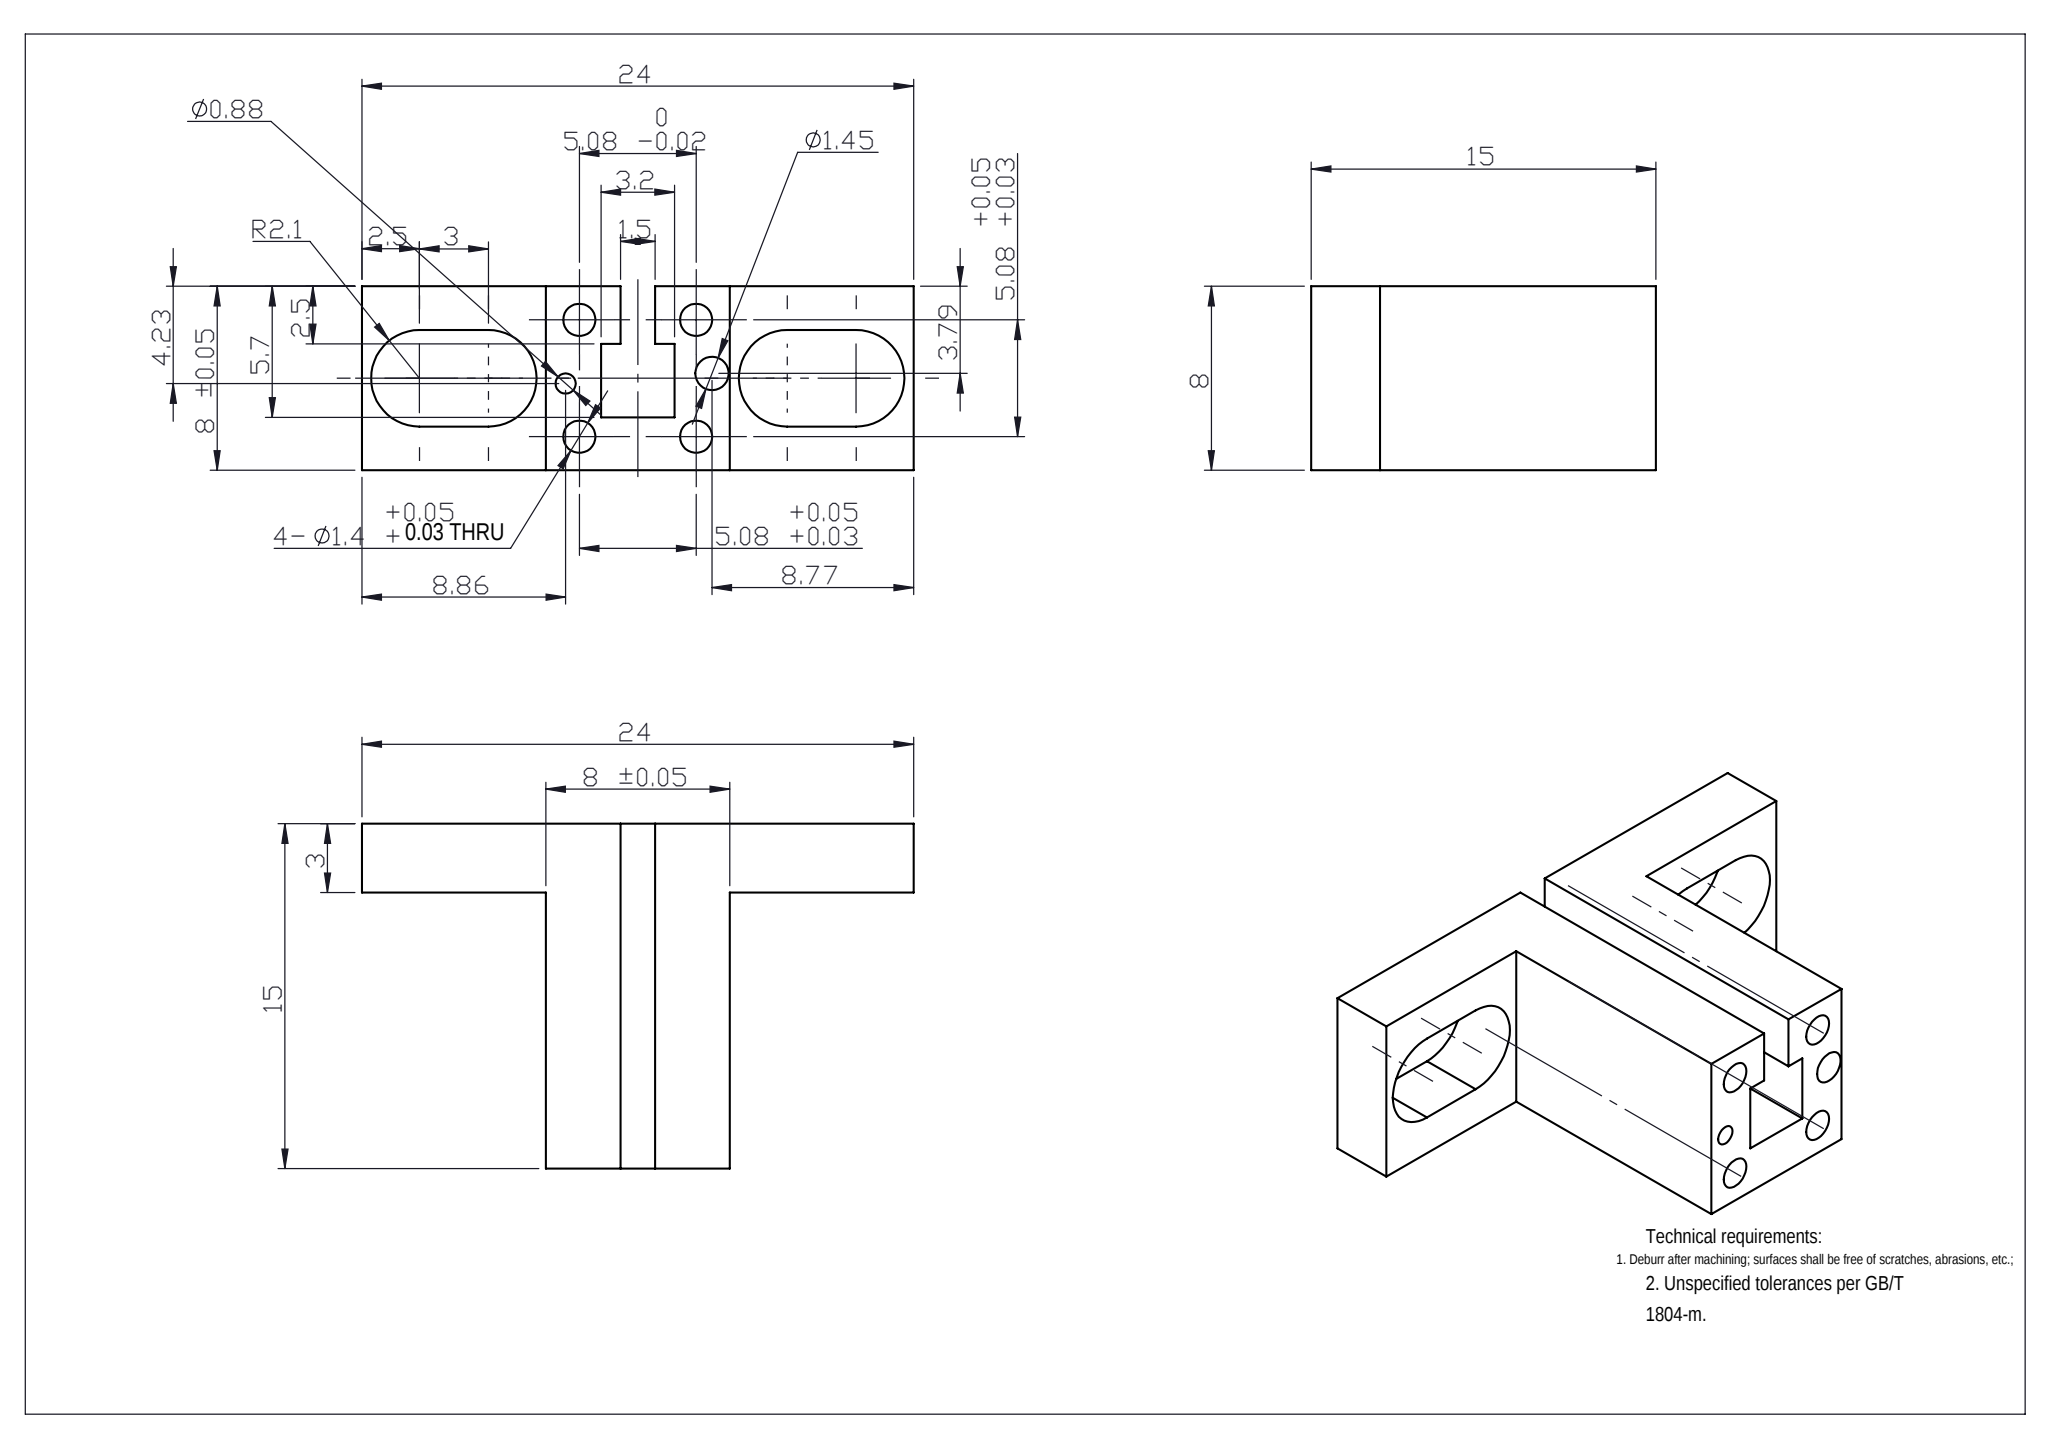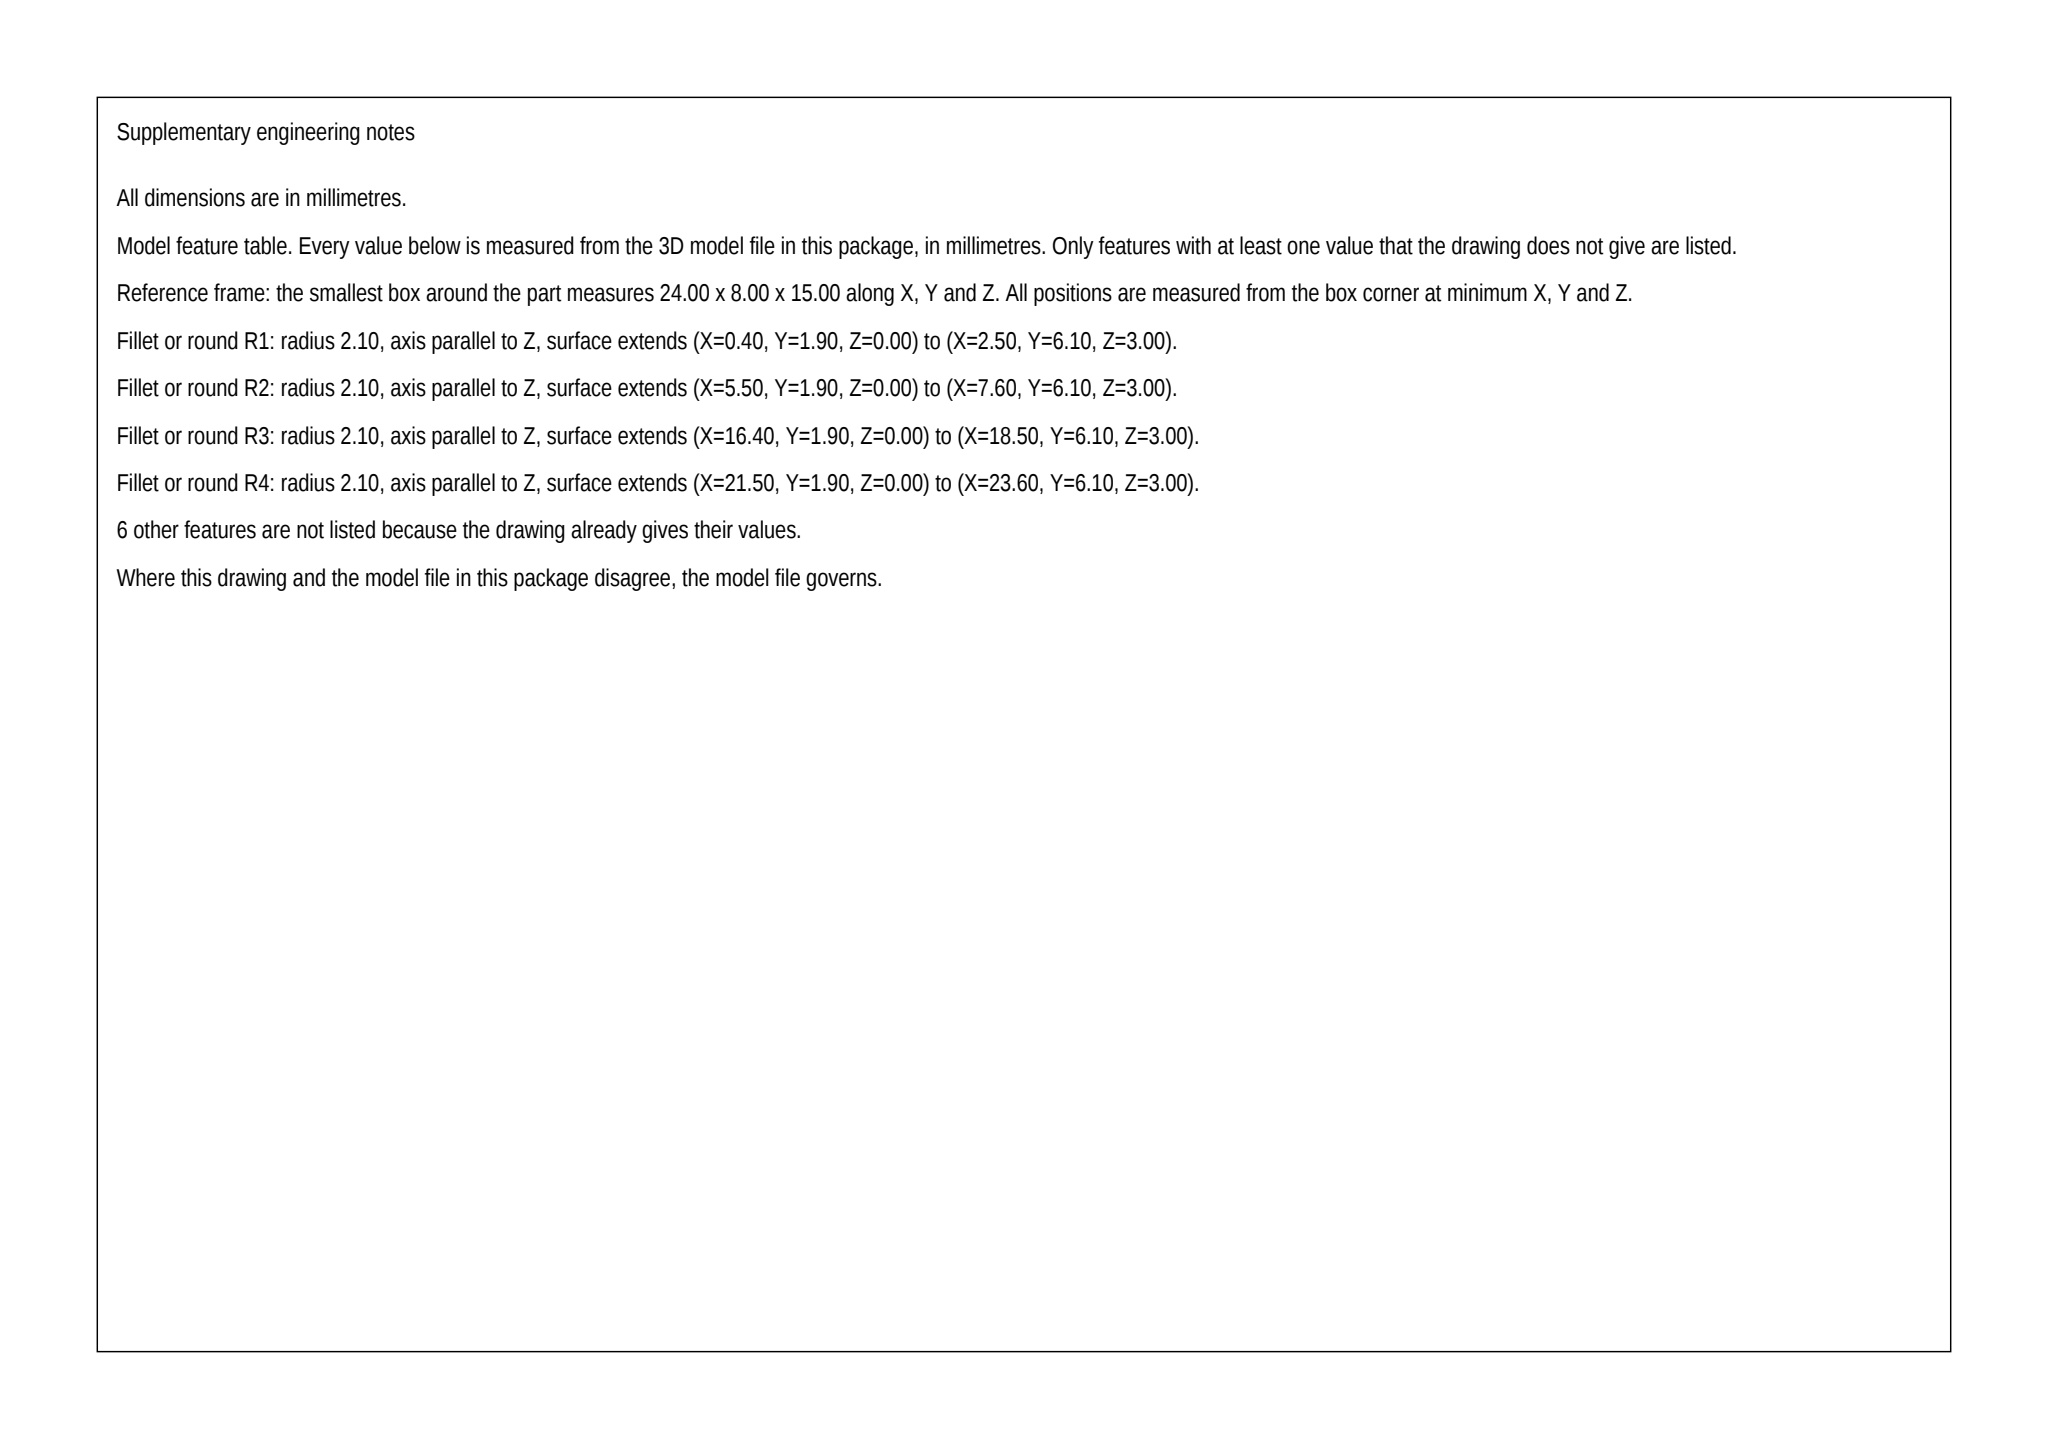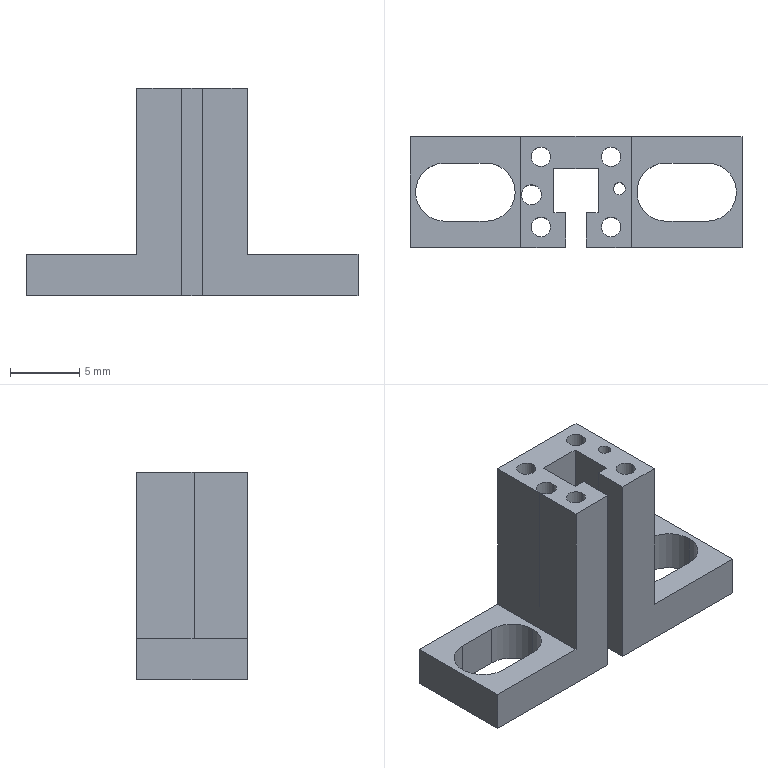Part | SolidWorks | mm | 1 solid | 40 faces | box 24 x 8 x 15 mm | volume 849 mm3 | plane 22 | cylinder 18 | commonest cylinder face diameters 1.4 x8 4.2 x6 0.879 x2 1.45 x2
build123d program:
from build123d import *

# Parameters (mm, degrees)
SKETCH1_W           = 8
SKETCH1_H           = 8
BOSS_EXTRUDE1_DEPTH = 15
SKETCH2_W           = 3
SKETCH2_H           = 8
BOSS_EXTRUDE2_DEPTH = 8
SKETCH3_W           = 3
SKETCH3_H           = 8
BOSS_EXTRUDE3_DEPTH = 8
CUT_EXTRUDE1_DEPTH  = 22.541
SKETCH7_R           = 0.7
CUT_EXTRUDE4_DEPTH  = 24.345
CUT_EXTRUDE5_DEPTH  = 24.345
SKETCH9_R           = 0.4393
SKETCH9_R_2         = 0.7249
CUT_EXTRUDE6_DEPTH  = 17


with BuildPart() as part:
    # Sketch1 → Boss-Extrude1 (new body)
    with BuildSketch(Plane.XY):
        with Locations((4, -4)):
            Rectangle(SKETCH1_W, SKETCH1_H)
    extrude(amount=BOSS_EXTRUDE1_DEPTH)

    # Sketch2 → Boss-Extrude2 (add)
    with BuildSketch(Plane(origin=(8, 0, 0), x_dir=(0, 0, -1), z_dir=(1, 0, 0))):
        with Locations((-1.5, -4)):
            Rectangle(SKETCH2_W, SKETCH2_H)
    extrude(amount=BOSS_EXTRUDE2_DEPTH)

    # Sketch3 → Boss-Extrude3 (add)
    with BuildSketch(Plane.ZY):
        with Locations((1.5, -4)):
            Rectangle(SKETCH3_W, SKETCH3_H)
    extrude(amount=BOSS_EXTRUDE3_DEPTH)

    # Sketch4 → Cut-Extrude1 (cut, through all)
    with BuildSketch(Plane.XY.offset(3)):
        with BuildLine():
            Line((-5.5, -1.9), (-2.5, -1.9))
            ThreePointArc((-2.5, -1.9), (-0.4, -4), (-2.5, -6.1))
            Line((-2.5, -6.1), (-5.5, -6.1))
            ThreePointArc((-5.5, -6.1), (-7.6, -4), (-5.5, -1.9))
        make_face()
        with BuildLine():
            Line((10.5, -1.9), (13.5, -1.9))
            ThreePointArc((13.5, -1.9), (15.6, -4), (13.5, -6.1))
            Line((13.5, -6.1), (10.5, -6.1))
            ThreePointArc((10.5, -6.1), (8.4, -4), (10.5, -1.9))
        make_face()
    extrude(amount=-CUT_EXTRUDE1_DEPTH, mode=Mode.SUBTRACT)

    # Sketch7 → Cut-Extrude4 (cut, through all)
    with BuildSketch(Plane.XY.offset(15)):
        with Locations((6.54, -6.54)):
            Circle(SKETCH7_R)
        with Locations((1.46, -6.54)):
            Circle(SKETCH7_R)
        with Locations((1.46, -1.46)):
            Circle(SKETCH7_R)
        with Locations((6.54, -1.46)):
            Circle(SKETCH7_R)
    extrude(amount=-CUT_EXTRUDE4_DEPTH, mode=Mode.SUBTRACT)

    # Sketch8 → Cut-Extrude5 (cut, through all)
    with BuildSketch(Plane.XY.offset(15)):
        Polygon((4.75, -8), (4.75, -5.5), (5.6, -5.5), (5.6, -2.3), (2.4, -2.3), (2.4, -5.5), (3.25, -5.5), (3.25, -8), align=None)
    extrude(amount=-CUT_EXTRUDE5_DEPTH, mode=Mode.SUBTRACT)

    # Sketch9 → Cut-Extrude6 (cut)
    with BuildSketch(Plane(origin=(0, 0, 0), x_dir=(-1, 0, 0), z_dir=(0, 0, -1))):
        with Locations((-7.137, -3.772)):
            Circle(SKETCH9_R)
        with Locations((-0.7713, -4.211)):
            Circle(SKETCH9_R_2)
    extrude(amount=-CUT_EXTRUDE6_DEPTH, mode=Mode.SUBTRACT)


solid = part.part